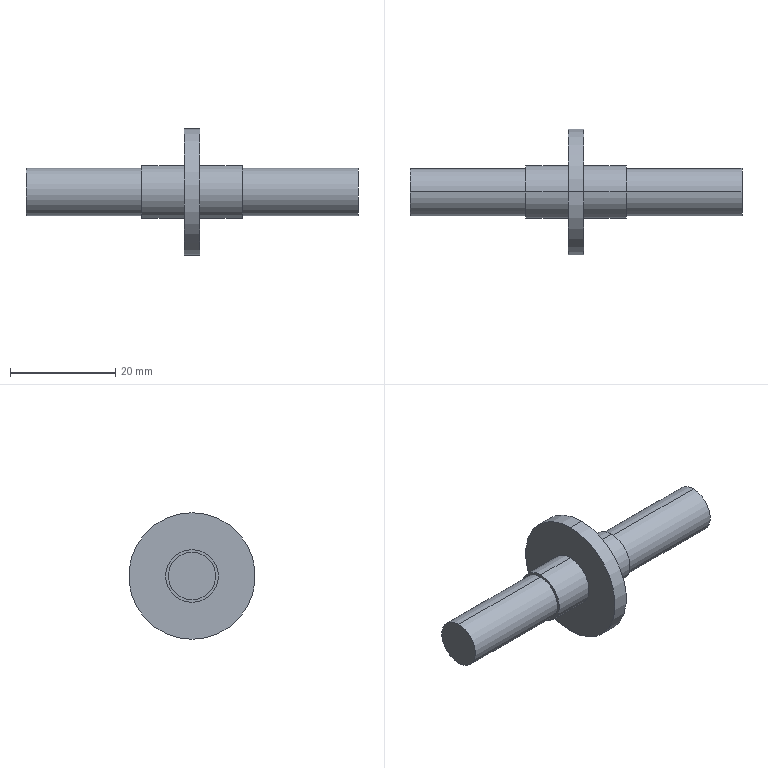Component | SolidWorks | RotatingShaft-1 | 1 solid | 16 faces | box 63 x 24 x 24 mm | volume 5413 mm3 | cylinder 10 | plane 6 | commonest cylinder face diameters 9 x4 10 x4 24 x2
STEP:
#1=COLOUR_RGB('',0.7922,0.8196,0.9333);
#2=FILL_AREA_STYLE_COLOUR('',#1);
#3=FILL_AREA_STYLE('',(#2));
#4=SURFACE_STYLE_FILL_AREA(#3);
#5=SURFACE_SIDE_STYLE('',(#4));
#6=SURFACE_STYLE_USAGE(.BOTH.,#5);
#7=PRESENTATION_STYLE_ASSIGNMENT((#6));
#8=CARTESIAN_POINT('',(8.268,2.91,9.227));
#9=VERTEX_POINT('',#8);
#10=CARTESIAN_POINT('',(8.268,2.91,8.872));
#11=VERTEX_POINT('',#10);
#12=CARTESIAN_POINT('',(8.268,2.91,9.049));
#13=DIRECTION('',(-1.,-0.,0.));
#14=DIRECTION('',(0.,-0.00000072,1.));
#15=AXIS2_PLACEMENT_3D('',#12,#13,#14);
#16=CIRCLE('',#15,0.1772);
#17=EDGE_CURVE('',#9,#11,#16,.T.);
#18=ORIENTED_EDGE('',*,*,#17,.F.);
#19=CARTESIAN_POINT('',(9.134,2.91,9.227));
#20=VERTEX_POINT('',#19);
#21=CARTESIAN_POINT('',(8.228,2.91,9.227));
#22=DIRECTION('',(1.,0.,-0.));
#23=VECTOR('',#22,39.37);
#24=LINE('',#21,#23);
#25=EDGE_CURVE('',#9,#20,#24,.T.);
#26=ORIENTED_EDGE('',*,*,#25,.T.);
#27=CARTESIAN_POINT('',(9.134,2.91,8.872));
#28=VERTEX_POINT('',#27);
#29=CARTESIAN_POINT('',(9.134,2.91,9.049));
#30=DIRECTION('',(1.,0.,-0.));
#31=DIRECTION('',(0.,0.00000072,-1.));
#32=AXIS2_PLACEMENT_3D('',#29,#30,#31);
#33=CIRCLE('',#32,0.1772);
#34=EDGE_CURVE('',#28,#20,#33,.T.);
#35=ORIENTED_EDGE('',*,*,#34,.F.);
#36=CARTESIAN_POINT('',(8.228,2.91,8.872));
#37=DIRECTION('',(1.,0.,-0.));
#38=VECTOR('',#37,39.37);
#39=LINE('',#36,#38);
#40=EDGE_CURVE('',#11,#28,#39,.T.);
#41=ORIENTED_EDGE('',*,*,#40,.F.);
#42=EDGE_LOOP('',(#18,#26,#35,#41));
#43=FACE_OUTER_BOUND('',#42,.T.);
#44=CARTESIAN_POINT('',(8.228,2.91,9.049));
#45=DIRECTION('',(1.,0.,-0.));
#46=DIRECTION('',(0.,0.00000072,-1.));
#47=AXIS2_PLACEMENT_3D('',#44,#45,#46);
#48=CYLINDRICAL_SURFACE('',#47,0.1772);
#49=ADVANCED_FACE('',(#43),#48,.T.);
#50=CARTESIAN_POINT('',(6.654,2.91,9.227));
#51=VERTEX_POINT('',#50);
#52=CARTESIAN_POINT('',(6.654,2.91,8.872));
#53=VERTEX_POINT('',#52);
#54=CARTESIAN_POINT('',(6.654,2.91,9.049));
#55=DIRECTION('',(-1.,-0.,0.));
#56=DIRECTION('',(0.,-0.00000072,1.));
#57=AXIS2_PLACEMENT_3D('',#54,#55,#56);
#58=CIRCLE('',#57,0.1772);
#59=EDGE_CURVE('',#51,#53,#58,.T.);
#60=ORIENTED_EDGE('',*,*,#59,.F.);
#61=CARTESIAN_POINT('',(7.52,2.91,9.227));
#62=VERTEX_POINT('',#61);
#63=CARTESIAN_POINT('',(6.594,2.91,9.227));
#64=DIRECTION('',(1.,0.,-0.));
#65=VECTOR('',#64,39.37);
#66=LINE('',#63,#65);
#67=EDGE_CURVE('',#51,#62,#66,.T.);
#68=ORIENTED_EDGE('',*,*,#67,.T.);
#69=CARTESIAN_POINT('',(7.52,2.91,8.872));
#70=VERTEX_POINT('',#69);
#71=CARTESIAN_POINT('',(7.52,2.91,9.049));
#72=DIRECTION('',(1.,0.,-0.));
#73=DIRECTION('',(0.,0.00000072,-1.));
#74=AXIS2_PLACEMENT_3D('',#71,#72,#73);
#75=CIRCLE('',#74,0.1772);
#76=EDGE_CURVE('',#70,#62,#75,.T.);
#77=ORIENTED_EDGE('',*,*,#76,.F.);
#78=CARTESIAN_POINT('',(6.594,2.91,8.872));
#79=DIRECTION('',(1.,0.,-0.));
#80=VECTOR('',#79,39.37);
#81=LINE('',#78,#80);
#82=EDGE_CURVE('',#53,#70,#81,.T.);
#83=ORIENTED_EDGE('',*,*,#82,.F.);
#84=EDGE_LOOP('',(#60,#68,#77,#83));
#85=FACE_OUTER_BOUND('',#84,.T.);
#86=CARTESIAN_POINT('',(6.594,2.91,9.049));
#87=DIRECTION('',(1.,0.,-0.));
#88=DIRECTION('',(0.,0.00000072,-1.));
#89=AXIS2_PLACEMENT_3D('',#86,#87,#88);
#90=CYLINDRICAL_SURFACE('',#89,0.1772);
#91=ADVANCED_FACE('',(#85),#90,.T.);
#92=CARTESIAN_POINT('',(7.52,2.91,9.246));
#93=VERTEX_POINT('',#92);
#94=CARTESIAN_POINT('',(7.52,2.91,8.853));
#95=VERTEX_POINT('',#94);
#96=CARTESIAN_POINT('',(7.52,2.91,9.049));
#97=DIRECTION('',(-1.,-0.,0.));
#98=DIRECTION('',(0.,0.00000072,-1.));
#99=AXIS2_PLACEMENT_3D('',#96,#97,#98);
#100=CIRCLE('',#99,0.1969);
#101=EDGE_CURVE('',#93,#95,#100,.T.);
#102=ORIENTED_EDGE('',*,*,#101,.F.);
#103=CARTESIAN_POINT('',(7.835,2.91,9.246));
#104=VERTEX_POINT('',#103);
#105=CARTESIAN_POINT('',(6.654,2.91,9.246));
#106=DIRECTION('',(1.,0.,-0.));
#107=VECTOR('',#106,39.37);
#108=LINE('',#105,#107);
#109=EDGE_CURVE('',#93,#104,#108,.T.);
#110=ORIENTED_EDGE('',*,*,#109,.T.);
#111=CARTESIAN_POINT('',(7.835,2.91,8.853));
#112=VERTEX_POINT('',#111);
#113=CARTESIAN_POINT('',(7.835,2.91,9.049));
#114=DIRECTION('',(1.,0.,-0.));
#115=DIRECTION('',(0.,0.00000072,-1.));
#116=AXIS2_PLACEMENT_3D('',#113,#114,#115);
#117=CIRCLE('',#116,0.1969);
#118=EDGE_CURVE('',#112,#104,#117,.T.);
#119=ORIENTED_EDGE('',*,*,#118,.F.);
#120=CARTESIAN_POINT('',(6.654,2.91,8.853));
#121=DIRECTION('',(1.,0.,-0.));
#122=VECTOR('',#121,39.37);
#123=LINE('',#120,#122);
#124=EDGE_CURVE('',#95,#112,#123,.T.);
#125=ORIENTED_EDGE('',*,*,#124,.F.);
#126=EDGE_LOOP('',(#102,#110,#119,#125));
#127=FACE_OUTER_BOUND('',#126,.T.);
#128=CARTESIAN_POINT('',(6.654,2.91,9.049));
#129=DIRECTION('',(1.,0.,-0.));
#130=DIRECTION('',(0.,0.00000072,-1.));
#131=AXIS2_PLACEMENT_3D('',#128,#129,#130);
#132=CYLINDRICAL_SURFACE('',#131,0.1969);
#133=ADVANCED_FACE('',(#127),#132,.T.);
#134=CARTESIAN_POINT('',(8.268,2.91,9.246));
#135=VERTEX_POINT('',#134);
#136=CARTESIAN_POINT('',(8.268,2.91,8.853));
#137=VERTEX_POINT('',#136);
#138=CARTESIAN_POINT('',(8.268,2.91,9.049));
#139=DIRECTION('',(-1.,-0.,0.));
#140=DIRECTION('',(0.,-0.00000072,1.));
#141=AXIS2_PLACEMENT_3D('',#138,#139,#140);
#142=CIRCLE('',#141,0.1969);
#143=EDGE_CURVE('',#135,#137,#142,.T.);
#144=ORIENTED_EDGE('',*,*,#143,.T.);
#145=CARTESIAN_POINT('',(7.953,2.91,8.853));
#146=VERTEX_POINT('',#145);
#147=CARTESIAN_POINT('',(9.134,2.91,8.853));
#148=DIRECTION('',(-1.,-0.,0.));
#149=VECTOR('',#148,39.37);
#150=LINE('',#147,#149);
#151=EDGE_CURVE('',#137,#146,#150,.T.);
#152=ORIENTED_EDGE('',*,*,#151,.T.);
#153=CARTESIAN_POINT('',(7.953,2.91,9.246));
#154=VERTEX_POINT('',#153);
#155=CARTESIAN_POINT('',(7.953,2.91,9.049));
#156=DIRECTION('',(1.,0.,-0.));
#157=DIRECTION('',(0.,0.00000072,-1.));
#158=AXIS2_PLACEMENT_3D('',#155,#156,#157);
#159=CIRCLE('',#158,0.1969);
#160=EDGE_CURVE('',#146,#154,#159,.T.);
#161=ORIENTED_EDGE('',*,*,#160,.T.);
#162=CARTESIAN_POINT('',(9.134,2.91,9.246));
#163=DIRECTION('',(-1.,-0.,0.));
#164=VECTOR('',#163,39.37);
#165=LINE('',#162,#164);
#166=EDGE_CURVE('',#135,#154,#165,.T.);
#167=ORIENTED_EDGE('',*,*,#166,.F.);
#168=EDGE_LOOP('',(#144,#152,#161,#167));
#169=FACE_OUTER_BOUND('',#168,.T.);
#170=CARTESIAN_POINT('',(9.134,2.91,9.049));
#171=DIRECTION('',(-1.,-0.,0.));
#172=DIRECTION('',(0.,-0.00000072,1.));
#173=AXIS2_PLACEMENT_3D('',#170,#171,#172);
#174=CYLINDRICAL_SURFACE('',#173,0.1969);
#175=ADVANCED_FACE('',(#169),#174,.T.);
#176=CARTESIAN_POINT('',(7.953,2.91,8.577));
#177=VERTEX_POINT('',#176);
#178=CARTESIAN_POINT('',(7.953,2.91,9.522));
#179=VERTEX_POINT('',#178);
#180=CARTESIAN_POINT('',(7.953,2.91,9.049));
#181=DIRECTION('',(1.,0.,-0.));
#182=DIRECTION('',(0.,0.00000072,-1.));
#183=AXIS2_PLACEMENT_3D('',#180,#181,#182);
#184=CIRCLE('',#183,0.4724);
#185=EDGE_CURVE('',#177,#179,#184,.T.);
#186=ORIENTED_EDGE('',*,*,#185,.F.);
#187=CARTESIAN_POINT('',(7.835,2.91,8.577));
#188=VERTEX_POINT('',#187);
#189=CARTESIAN_POINT('',(7.953,2.91,8.577));
#190=DIRECTION('',(-1.,-0.,0.));
#191=VECTOR('',#190,39.37);
#192=LINE('',#189,#191);
#193=EDGE_CURVE('',#177,#188,#192,.T.);
#194=ORIENTED_EDGE('',*,*,#193,.T.);
#195=CARTESIAN_POINT('',(7.835,2.91,9.522));
#196=VERTEX_POINT('',#195);
#197=CARTESIAN_POINT('',(7.835,2.91,9.049));
#198=DIRECTION('',(1.,0.,-0.));
#199=DIRECTION('',(0.,0.00000072,-1.));
#200=AXIS2_PLACEMENT_3D('',#197,#198,#199);
#201=CIRCLE('',#200,0.4724);
#202=EDGE_CURVE('',#188,#196,#201,.T.);
#203=ORIENTED_EDGE('',*,*,#202,.T.);
#204=CARTESIAN_POINT('',(7.953,2.91,9.522));
#205=DIRECTION('',(-1.,-0.,0.));
#206=VECTOR('',#205,39.37);
#207=LINE('',#204,#206);
#208=EDGE_CURVE('',#179,#196,#207,.T.);
#209=ORIENTED_EDGE('',*,*,#208,.F.);
#210=EDGE_LOOP('',(#186,#194,#203,#209));
#211=FACE_OUTER_BOUND('',#210,.T.);
#212=CARTESIAN_POINT('',(7.953,2.91,9.049));
#213=DIRECTION('',(-1.,-0.,0.));
#214=DIRECTION('',(0.,-0.00000072,1.));
#215=AXIS2_PLACEMENT_3D('',#212,#213,#214);
#216=CYLINDRICAL_SURFACE('',#215,0.4724);
#217=ADVANCED_FACE('',(#211),#216,.T.);
#218=CARTESIAN_POINT('',(7.953,2.91,9.049));
#219=DIRECTION('',(1.,0.,-0.));
#220=DIRECTION('',(0.,0.00000072,-1.));
#221=AXIS2_PLACEMENT_3D('',#218,#219,#220);
#222=CIRCLE('',#221,0.4724);
#223=EDGE_CURVE('',#179,#177,#222,.T.);
#224=ORIENTED_EDGE('',*,*,#223,.T.);
#225=ORIENTED_EDGE('',*,*,#185,.T.);
#226=EDGE_LOOP('',(#224,#225));
#227=FACE_OUTER_BOUND('',#226,.T.);
#228=CARTESIAN_POINT('',(7.953,2.91,9.049));
#229=DIRECTION('',(1.,0.,-0.));
#230=DIRECTION('',(0.,0.00000072,-1.));
#231=AXIS2_PLACEMENT_3D('',#228,#229,#230);
#232=CIRCLE('',#231,0.1969);
#233=EDGE_CURVE('',#154,#146,#232,.T.);
#234=ORIENTED_EDGE('',*,*,#233,.F.);
#235=ORIENTED_EDGE('',*,*,#160,.F.);
#236=EDGE_LOOP('',(#234,#235));
#237=FACE_BOUND('',#236,.T.);
#238=CARTESIAN_POINT('',(7.953,2.91,9.049));
#239=DIRECTION('',(1.,0.,-0.));
#240=DIRECTION('',(-0.,0.00000072,-1.));
#241=AXIS2_PLACEMENT_3D('',#238,#239,#240);
#242=PLANE('',#241);
#243=ADVANCED_FACE('',(#227,#237),#242,.T.);
#244=ORIENTED_EDGE('',*,*,#193,.F.);
#245=ORIENTED_EDGE('',*,*,#223,.F.);
#246=ORIENTED_EDGE('',*,*,#208,.T.);
#247=CARTESIAN_POINT('',(7.835,2.91,9.049));
#248=DIRECTION('',(1.,0.,-0.));
#249=DIRECTION('',(0.,0.00000072,-1.));
#250=AXIS2_PLACEMENT_3D('',#247,#248,#249);
#251=CIRCLE('',#250,0.4724);
#252=EDGE_CURVE('',#196,#188,#251,.T.);
#253=ORIENTED_EDGE('',*,*,#252,.T.);
#254=EDGE_LOOP('',(#244,#245,#246,#253));
#255=FACE_OUTER_BOUND('',#254,.T.);
#256=CARTESIAN_POINT('',(7.953,2.91,9.049));
#257=DIRECTION('',(-1.,-0.,0.));
#258=DIRECTION('',(0.,-0.00000072,1.));
#259=AXIS2_PLACEMENT_3D('',#256,#257,#258);
#260=CYLINDRICAL_SURFACE('',#259,0.4724);
#261=ADVANCED_FACE('',(#255),#260,.T.);
#262=ORIENTED_EDGE('',*,*,#118,.T.);
#263=CARTESIAN_POINT('',(7.835,2.91,9.049));
#264=DIRECTION('',(1.,0.,-0.));
#265=DIRECTION('',(0.,0.00000072,-1.));
#266=AXIS2_PLACEMENT_3D('',#263,#264,#265);
#267=CIRCLE('',#266,0.1969);
#268=EDGE_CURVE('',#104,#112,#267,.T.);
#269=ORIENTED_EDGE('',*,*,#268,.T.);
#270=EDGE_LOOP('',(#262,#269));
#271=FACE_BOUND('',#270,.T.);
#272=ORIENTED_EDGE('',*,*,#252,.F.);
#273=ORIENTED_EDGE('',*,*,#202,.F.);
#274=EDGE_LOOP('',(#272,#273));
#275=FACE_OUTER_BOUND('',#274,.T.);
#276=CARTESIAN_POINT('',(7.835,2.91,9.049));
#277=DIRECTION('',(1.,0.,-0.));
#278=DIRECTION('',(-0.,0.00000072,-1.));
#279=AXIS2_PLACEMENT_3D('',#276,#277,#278);
#280=PLANE('',#279);
#281=ADVANCED_FACE('',(#271,#275),#280,.F.);
#282=ORIENTED_EDGE('',*,*,#151,.F.);
#283=CARTESIAN_POINT('',(8.268,2.91,9.049));
#284=DIRECTION('',(-1.,-0.,0.));
#285=DIRECTION('',(0.,-0.00000072,1.));
#286=AXIS2_PLACEMENT_3D('',#283,#284,#285);
#287=CIRCLE('',#286,0.1969);
#288=EDGE_CURVE('',#137,#135,#287,.T.);
#289=ORIENTED_EDGE('',*,*,#288,.T.);
#290=ORIENTED_EDGE('',*,*,#166,.T.);
#291=ORIENTED_EDGE('',*,*,#233,.T.);
#292=EDGE_LOOP('',(#282,#289,#290,#291));
#293=FACE_OUTER_BOUND('',#292,.T.);
#294=CARTESIAN_POINT('',(9.134,2.91,9.049));
#295=DIRECTION('',(-1.,-0.,0.));
#296=DIRECTION('',(0.,-0.00000072,1.));
#297=AXIS2_PLACEMENT_3D('',#294,#295,#296);
#298=CYLINDRICAL_SURFACE('',#297,0.1969);
#299=ADVANCED_FACE('',(#293),#298,.T.);
#300=ORIENTED_EDGE('',*,*,#109,.F.);
#301=CARTESIAN_POINT('',(7.52,2.91,9.049));
#302=DIRECTION('',(-1.,-0.,0.));
#303=DIRECTION('',(0.,0.00000072,-1.));
#304=AXIS2_PLACEMENT_3D('',#301,#302,#303);
#305=CIRCLE('',#304,0.1969);
#306=EDGE_CURVE('',#95,#93,#305,.T.);
#307=ORIENTED_EDGE('',*,*,#306,.F.);
#308=ORIENTED_EDGE('',*,*,#124,.T.);
#309=ORIENTED_EDGE('',*,*,#268,.F.);
#310=EDGE_LOOP('',(#300,#307,#308,#309));
#311=FACE_OUTER_BOUND('',#310,.T.);
#312=CARTESIAN_POINT('',(6.654,2.91,9.049));
#313=DIRECTION('',(1.,0.,-0.));
#314=DIRECTION('',(0.,0.00000072,-1.));
#315=AXIS2_PLACEMENT_3D('',#312,#313,#314);
#316=CYLINDRICAL_SURFACE('',#315,0.1969);
#317=ADVANCED_FACE('',(#311),#316,.T.);
#318=ORIENTED_EDGE('',*,*,#306,.T.);
#319=ORIENTED_EDGE('',*,*,#101,.T.);
#320=EDGE_LOOP('',(#318,#319));
#321=FACE_OUTER_BOUND('',#320,.T.);
#322=ORIENTED_EDGE('',*,*,#76,.T.);
#323=CARTESIAN_POINT('',(7.52,2.91,9.049));
#324=DIRECTION('',(1.,0.,-0.));
#325=DIRECTION('',(0.,0.00000072,-1.));
#326=AXIS2_PLACEMENT_3D('',#323,#324,#325);
#327=CIRCLE('',#326,0.1772);
#328=EDGE_CURVE('',#62,#70,#327,.T.);
#329=ORIENTED_EDGE('',*,*,#328,.T.);
#330=EDGE_LOOP('',(#322,#329));
#331=FACE_BOUND('',#330,.T.);
#332=CARTESIAN_POINT('',(7.52,2.91,9.049));
#333=DIRECTION('',(1.,0.,-0.));
#334=DIRECTION('',(-0.,0.00000072,-1.));
#335=AXIS2_PLACEMENT_3D('',#332,#333,#334);
#336=PLANE('',#335);
#337=ADVANCED_FACE('',(#321,#331),#336,.F.);
#338=ORIENTED_EDGE('',*,*,#67,.F.);
#339=CARTESIAN_POINT('',(6.654,2.91,9.049));
#340=DIRECTION('',(-1.,-0.,0.));
#341=DIRECTION('',(0.,-0.00000072,1.));
#342=AXIS2_PLACEMENT_3D('',#339,#340,#341);
#343=CIRCLE('',#342,0.1772);
#344=EDGE_CURVE('',#53,#51,#343,.T.);
#345=ORIENTED_EDGE('',*,*,#344,.F.);
#346=ORIENTED_EDGE('',*,*,#82,.T.);
#347=ORIENTED_EDGE('',*,*,#328,.F.);
#348=EDGE_LOOP('',(#338,#345,#346,#347));
#349=FACE_OUTER_BOUND('',#348,.T.);
#350=CARTESIAN_POINT('',(6.594,2.91,9.049));
#351=DIRECTION('',(1.,0.,-0.));
#352=DIRECTION('',(0.,0.00000072,-1.));
#353=AXIS2_PLACEMENT_3D('',#350,#351,#352);
#354=CYLINDRICAL_SURFACE('',#353,0.1772);
#355=ADVANCED_FACE('',(#349),#354,.T.);
#356=CARTESIAN_POINT('',(8.268,2.91,9.049));
#357=DIRECTION('',(-1.,-0.,0.));
#358=DIRECTION('',(0.,-0.00000072,1.));
#359=AXIS2_PLACEMENT_3D('',#356,#357,#358);
#360=CIRCLE('',#359,0.1772);
#361=EDGE_CURVE('',#11,#9,#360,.T.);
#362=ORIENTED_EDGE('',*,*,#361,.T.);
#363=ORIENTED_EDGE('',*,*,#17,.T.);
#364=EDGE_LOOP('',(#362,#363));
#365=FACE_BOUND('',#364,.T.);
#366=ORIENTED_EDGE('',*,*,#143,.F.);
#367=ORIENTED_EDGE('',*,*,#288,.F.);
#368=EDGE_LOOP('',(#366,#367));
#369=FACE_OUTER_BOUND('',#368,.T.);
#370=CARTESIAN_POINT('',(8.268,2.91,9.049));
#371=DIRECTION('',(-1.,-0.,0.));
#372=DIRECTION('',(0.,-0.00000072,1.));
#373=AXIS2_PLACEMENT_3D('',#370,#371,#372);
#374=PLANE('',#373);
#375=ADVANCED_FACE('',(#365,#369),#374,.F.);
#376=ORIENTED_EDGE('',*,*,#25,.F.);
#377=ORIENTED_EDGE('',*,*,#361,.F.);
#378=ORIENTED_EDGE('',*,*,#40,.T.);
#379=CARTESIAN_POINT('',(9.134,2.91,9.049));
#380=DIRECTION('',(1.,0.,-0.));
#381=DIRECTION('',(0.,0.00000072,-1.));
#382=AXIS2_PLACEMENT_3D('',#379,#380,#381);
#383=CIRCLE('',#382,0.1772);
#384=EDGE_CURVE('',#20,#28,#383,.T.);
#385=ORIENTED_EDGE('',*,*,#384,.F.);
#386=EDGE_LOOP('',(#376,#377,#378,#385));
#387=FACE_OUTER_BOUND('',#386,.T.);
#388=CARTESIAN_POINT('',(8.228,2.91,9.049));
#389=DIRECTION('',(1.,0.,-0.));
#390=DIRECTION('',(0.,0.00000072,-1.));
#391=AXIS2_PLACEMENT_3D('',#388,#389,#390);
#392=CYLINDRICAL_SURFACE('',#391,0.1772);
#393=ADVANCED_FACE('',(#387),#392,.T.);
#394=ORIENTED_EDGE('',*,*,#344,.T.);
#395=ORIENTED_EDGE('',*,*,#59,.T.);
#396=EDGE_LOOP('',(#394,#395));
#397=FACE_OUTER_BOUND('',#396,.T.);
#398=CARTESIAN_POINT('',(6.654,2.91,9.049));
#399=DIRECTION('',(-1.,-0.,0.));
#400=DIRECTION('',(-0.,0.00000072,-1.));
#401=AXIS2_PLACEMENT_3D('',#398,#399,#400);
#402=PLANE('',#401);
#403=ADVANCED_FACE('',(#397),#402,.T.);
#404=ORIENTED_EDGE('',*,*,#34,.T.);
#405=ORIENTED_EDGE('',*,*,#384,.T.);
#406=EDGE_LOOP('',(#404,#405));
#407=FACE_OUTER_BOUND('',#406,.T.);
#408=CARTESIAN_POINT('',(9.134,2.91,9.049));
#409=DIRECTION('',(1.,0.,-0.));
#410=DIRECTION('',(-0.,0.00000072,-1.));
#411=AXIS2_PLACEMENT_3D('',#408,#409,#410);
#412=PLANE('',#411);
#413=ADVANCED_FACE('',(#407),#412,.T.);
#414=CLOSED_SHELL('',(#49,#91,#133,#175,#217,#243,#261,#281,#299,#317,#337,#355,#375,#393,#403,#413));
#415=MANIFOLD_SOLID_BREP('',#414);
#416=STYLED_ITEM('',(#7),#415);
#417=PRESENTATION_LAYER_ASSIGNMENT('','',(#416));
#418=(LENGTH_UNIT()NAMED_UNIT(*)SI_UNIT($,.METRE.));
#419=LENGTH_MEASURE_WITH_UNIT(LENGTH_MEASURE(0.0254),#418);
#420=DIMENSIONAL_EXPONENTS(1.,0.,0.,0.,0.,0.,0.);
#421=(CONVERSION_BASED_UNIT('',#419)LENGTH_UNIT()NAMED_UNIT(#420));
#422=UNCERTAINTY_MEASURE_WITH_UNIT(LENGTH_MEASURE(0.00001),#421,'','');
#423=(NAMED_UNIT(*)PLANE_ANGLE_UNIT()SI_UNIT($,.RADIAN.));
#424=(NAMED_UNIT(*)SI_UNIT($,.STERADIAN.)SOLID_ANGLE_UNIT());
#425=(GEOMETRIC_REPRESENTATION_CONTEXT(3)GLOBAL_UNCERTAINTY_ASSIGNED_CONTEXT((#422))GLOBAL_UNIT_ASSIGNED_CONTEXT((#421,#423,#424))REPRESENTATION_CONTEXT('',''));
#426=MECHANICAL_DESIGN_GEOMETRIC_PRESENTATION_REPRESENTATION('',(#416),#425);
#427=CARTESIAN_POINT('',(0.,0.,0.));
#428=DIRECTION('',(0.,0.,1.));
#429=DIRECTION('',(1.,0.,0.));
#430=AXIS2_PLACEMENT_3D('',#427,#428,#429);
#431=(LENGTH_UNIT()NAMED_UNIT(*)SI_UNIT($,.METRE.));
#432=LENGTH_MEASURE_WITH_UNIT(LENGTH_MEASURE(0.0254),#431);
#433=DIMENSIONAL_EXPONENTS(1.,0.,0.,0.,0.,0.,0.);
#434=(CONVERSION_BASED_UNIT('',#432)LENGTH_UNIT()NAMED_UNIT(#433));
#435=UNCERTAINTY_MEASURE_WITH_UNIT(LENGTH_MEASURE(0.00001),#434,'','');
#436=(NAMED_UNIT(*)PLANE_ANGLE_UNIT()SI_UNIT($,.RADIAN.));
#437=(NAMED_UNIT(*)SI_UNIT($,.STERADIAN.)SOLID_ANGLE_UNIT());
#438=(GEOMETRIC_REPRESENTATION_CONTEXT(3)GLOBAL_UNCERTAINTY_ASSIGNED_CONTEXT((#435))GLOBAL_UNIT_ASSIGNED_CONTEXT((#434,#436,#437))REPRESENTATION_CONTEXT('',''));
#439=ADVANCED_BREP_SHAPE_REPRESENTATION('',(#415,#430),#438);